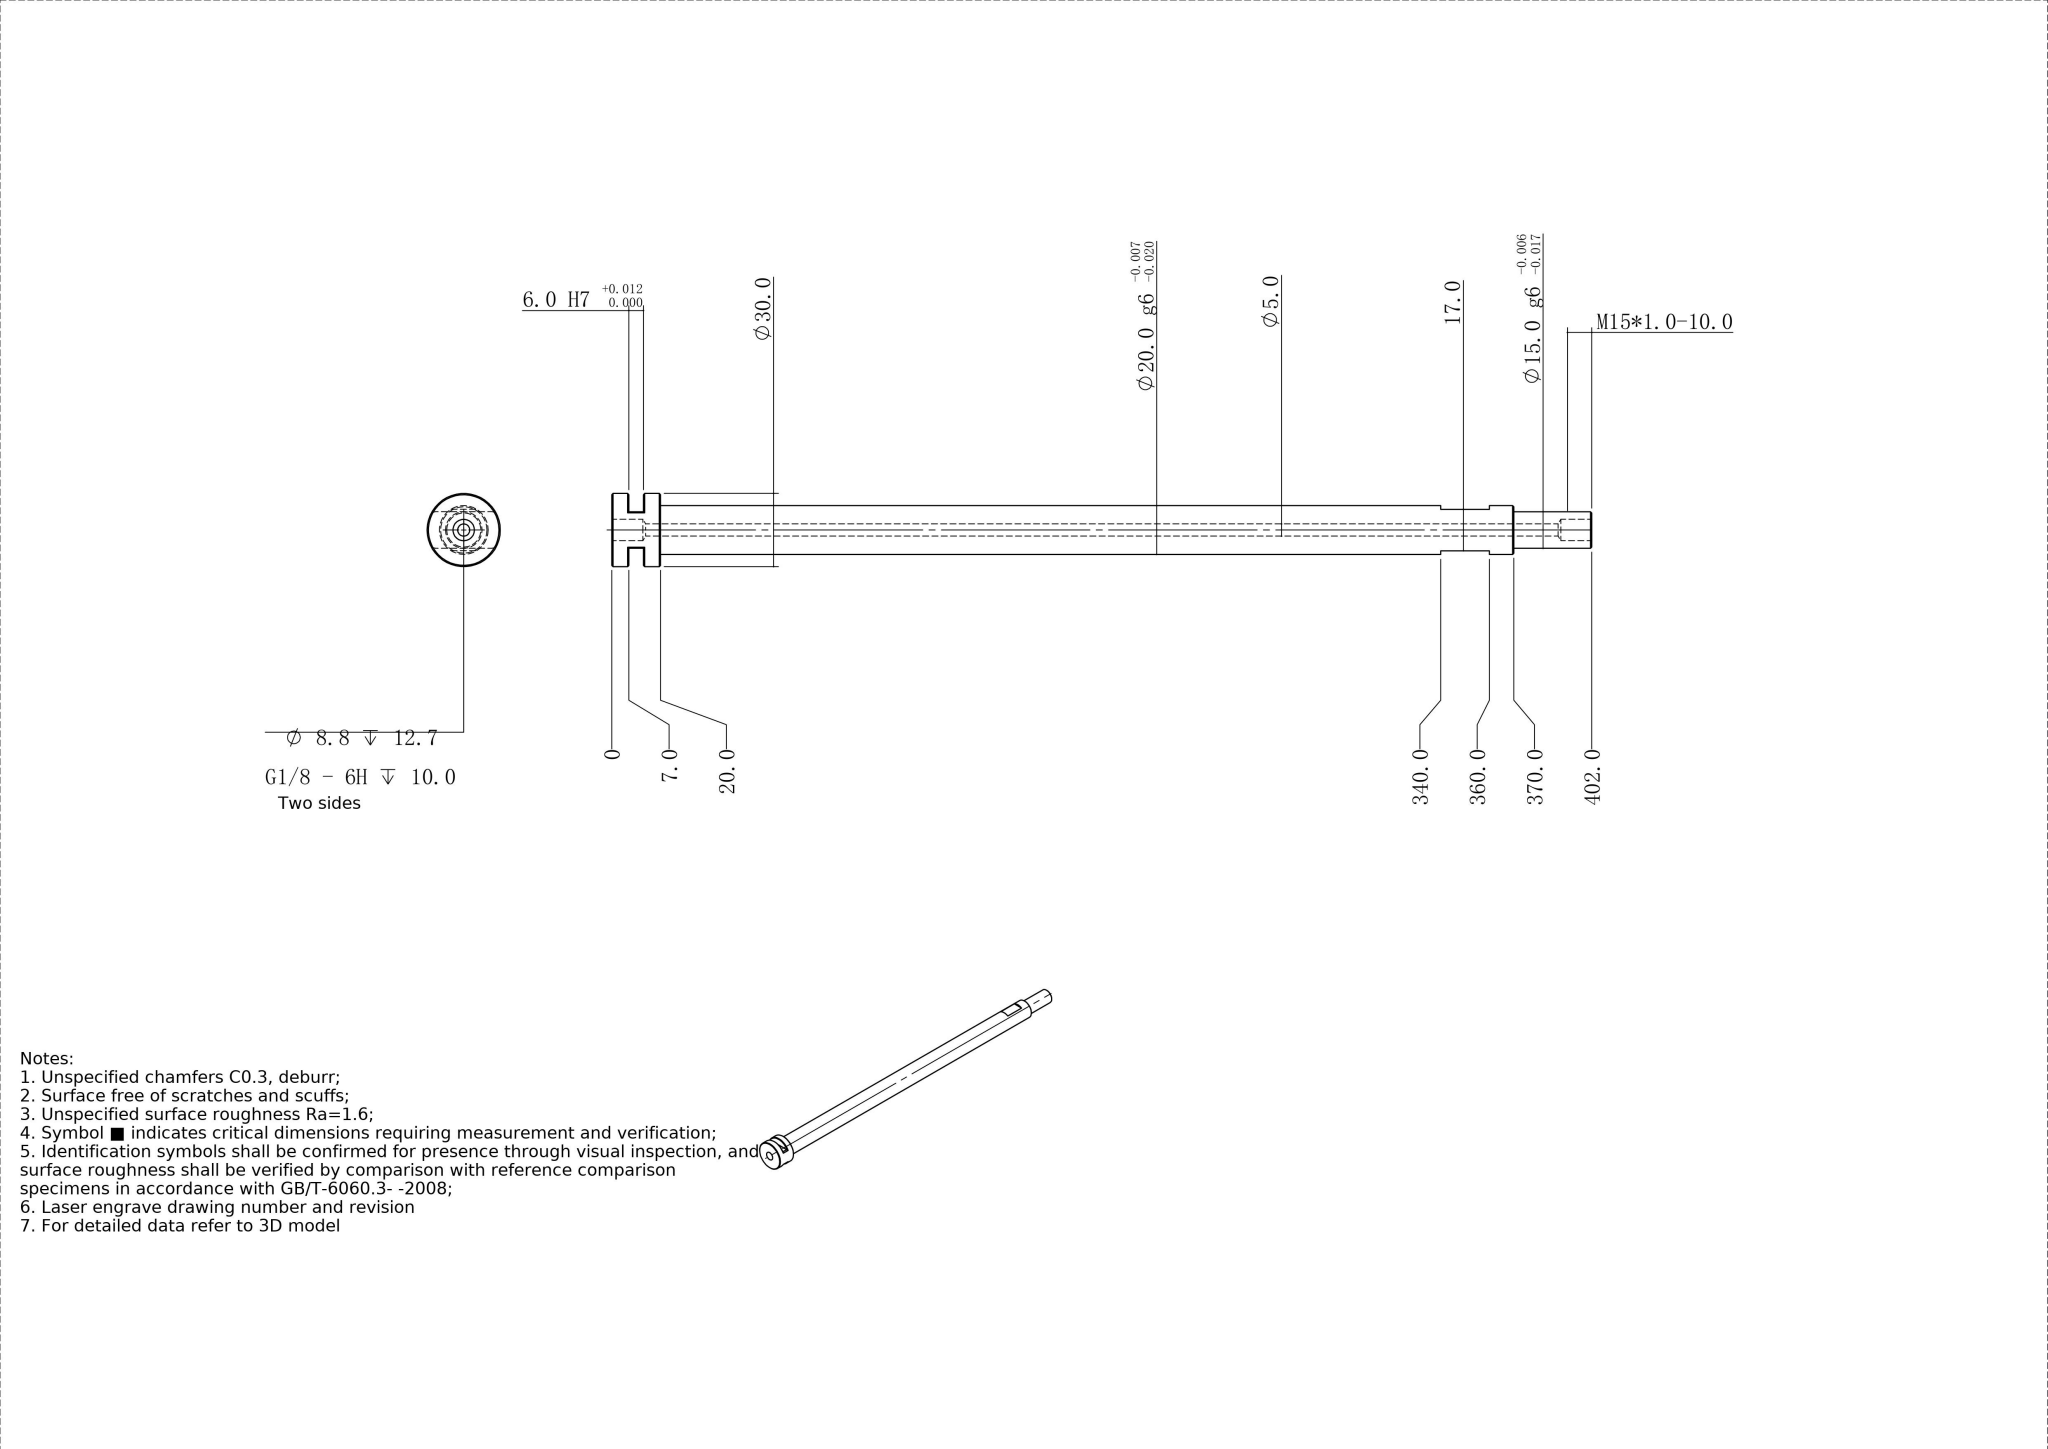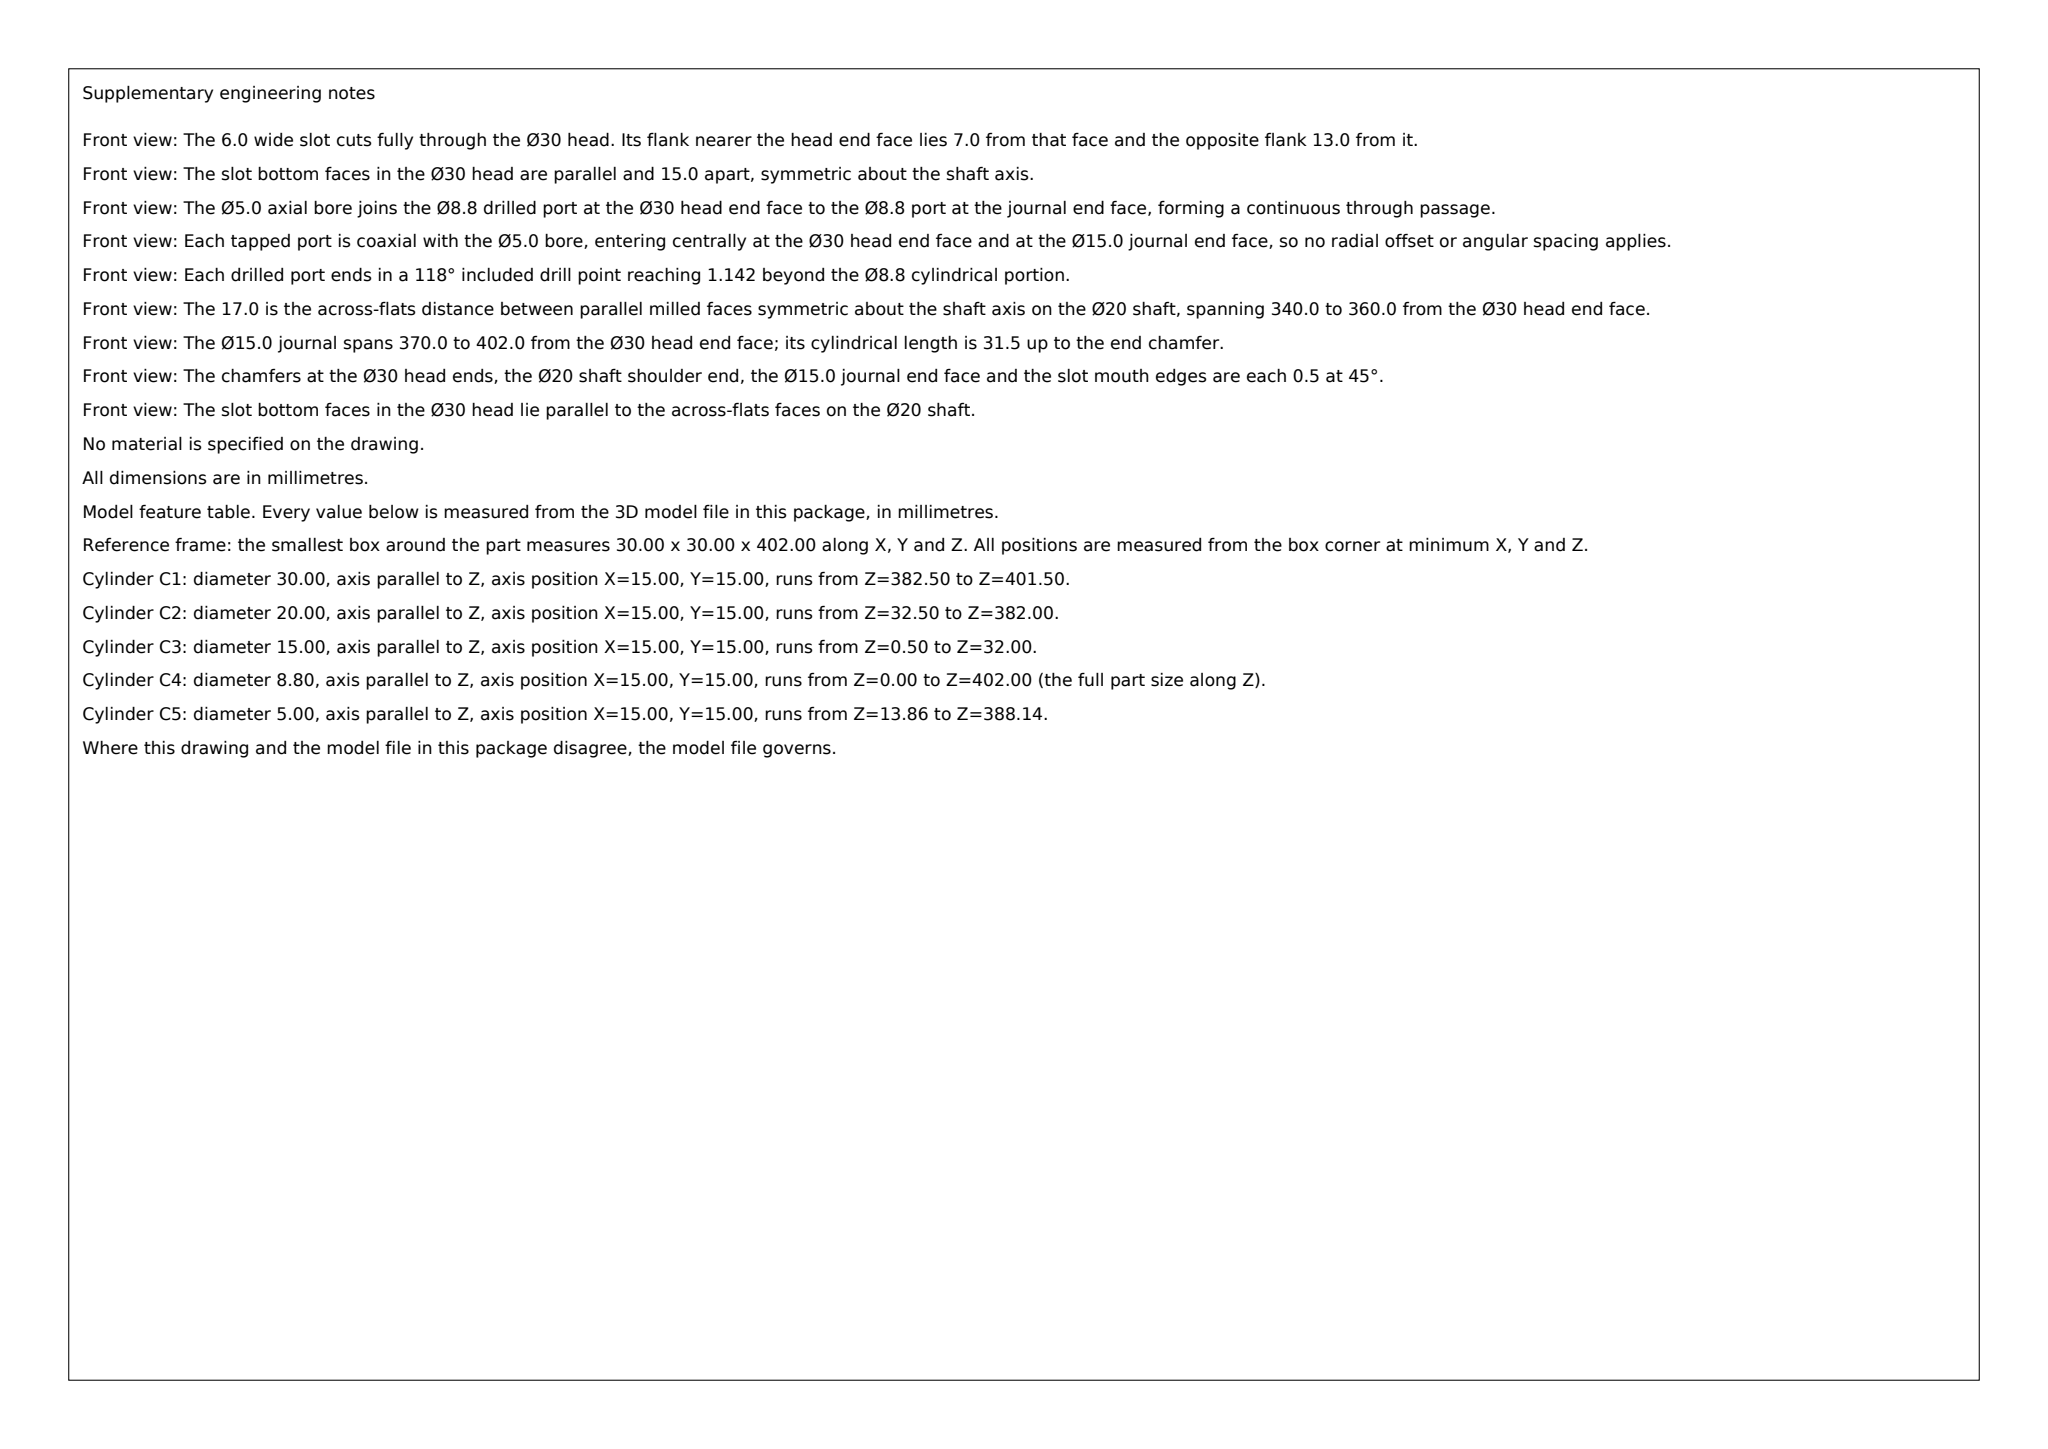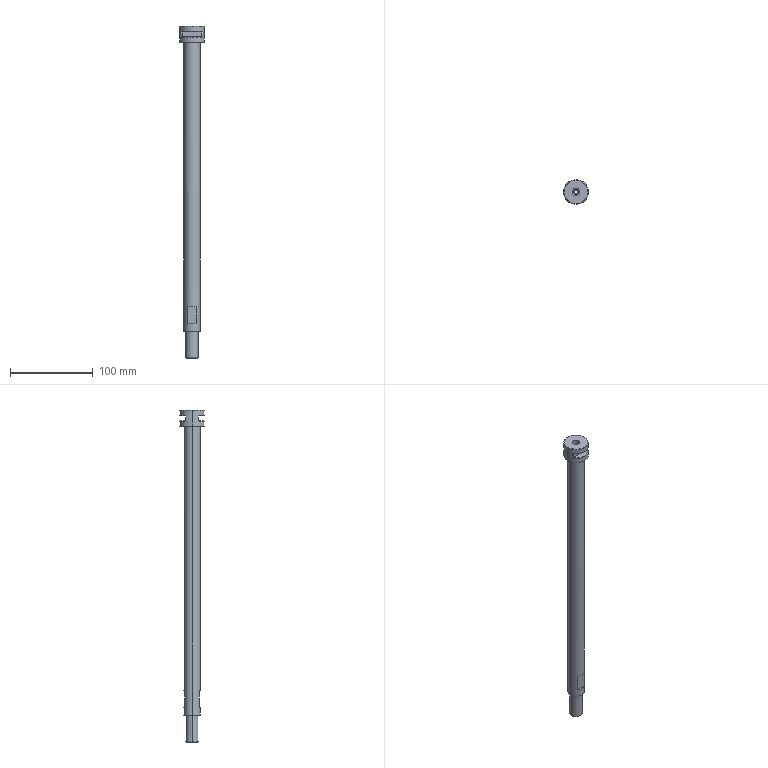Part | SolidWorks | mm | 1 solid | 48 faces | box 30 x 30 x 402 mm | volume 118618 mm3 | plane 20 | cone 16 | cylinder 12 | commonest cylinder face diameters 8.8 x4 30 x2 5 x2 15 x2 20 x2